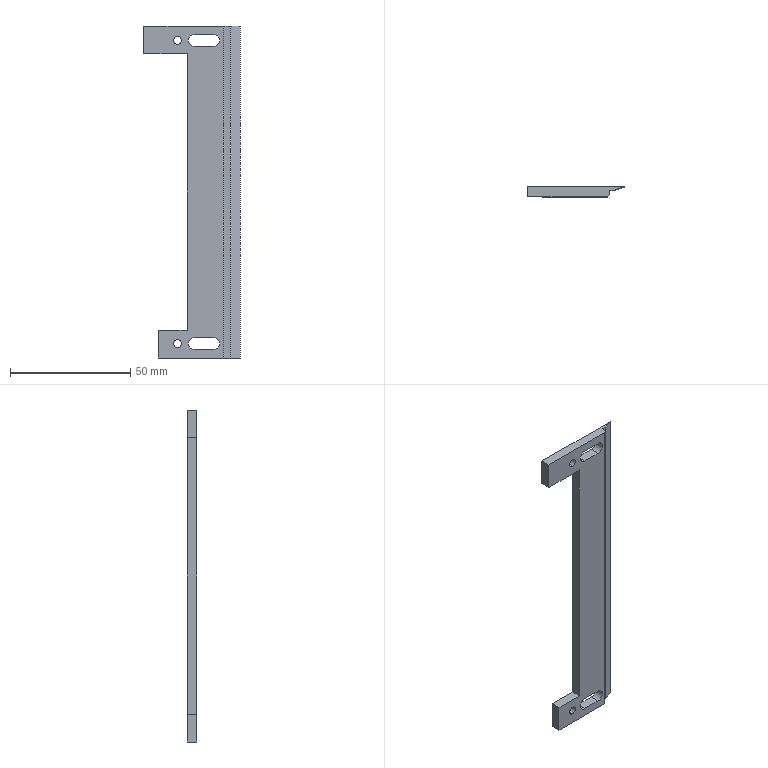Component | SolidWorks | FrameCutterBackingPlate.1-1 | 1 solid | 25 faces | box 40 x 4 x 138 mm | volume 10315 mm3 | plane 17 | cylinder 8 | commonest cylinder face diameters 3.3 x4 5 x4
build123d program:
from build123d import *

# Parameters (mm, degrees)
BOSS_EXTRUDE1_DEPTH   = 4
M4_TAPPED_HOLE1_D     = 3.3
M4_TAPPED_HOLE1_DEPTH = 10.1
M4_TAPPED_HOLE1_TIP   = 0.9914
CUT_EXTRUDE6_DEPTH    = 86.5
CHAMFER1_SIZE         = 1


with BuildPart() as part:
    # Sketch1 → Boss-Extrude1 (new body)
    with BuildSketch(Plane.XY):
        Polygon((-69, 41.921), (69, 41.921), (69, 1.921), (57.5, 1.921), (57.5, 19.921), (-57.5, 19.921), (-57.5, 7.921), (-69, 7.921), align=None)
        with BuildLine():
            Line((-60.5, 30.921), (-60.5, 22.921))
            ThreePointArc((-60.5, 22.921), (-63, 20.421), (-65.5, 22.921))
            Line((-65.5, 22.921), (-65.5, 30.921))
            ThreePointArc((-65.5, 30.921), (-63, 33.421), (-60.5, 30.921))
        make_face(mode=Mode.SUBTRACT)
        with BuildLine():
            Line((65.5, 30.921), (65.5, 22.921))
            ThreePointArc((65.5, 22.921), (63, 20.421), (60.5, 22.921))
            Line((60.5, 22.921), (60.5, 30.921))
            ThreePointArc((60.5, 30.921), (63, 33.421), (65.5, 30.921))
        make_face(mode=Mode.SUBTRACT)
    extrude(amount=BOSS_EXTRUDE1_DEPTH)

    # M4 Tapped Hole1
    with Locations(Plane(origin=(0, 0, 0), x_dir=(-1, 0, 0), z_dir=(0, 0, -1))):
        with Locations((-63, 15.921), (63, 15.921)):
            Hole(M4_TAPPED_HOLE1_D / 2, depth=M4_TAPPED_HOLE1_DEPTH)
            with Locations((0, 0, -(M4_TAPPED_HOLE1_DEPTH + M4_TAPPED_HOLE1_TIP / 2))):  # 118° drill point
                Cone(0, M4_TAPPED_HOLE1_D / 2, M4_TAPPED_HOLE1_TIP, mode=Mode.SUBTRACT)

    # Sketch2 → Cut-Extrude6 (cut, symmetric)
    with BuildSketch(Plane(origin=(0, 0, 0), x_dir=(0, 0, -1), z_dir=(1, 0, 0))):
        Polygon((1.372, 35.921), (-2.7, 35.921), (-2.7, 37.921), (-4, 41.921), (-4, 43.097), (1.372, 43.097), align=None)
    extrude(amount=CUT_EXTRUDE6_DEPTH, both=True, mode=Mode.SUBTRACT)

    # Chamfer1
    chamfer1_edges = [part.edges().sort_by_distance(p)[0] for p in [
        (0, 35.921, 0),
    ]]
    chamfer(chamfer1_edges, length=CHAMFER1_SIZE)


solid = part.part

# Placed as in the assembly
solid = solid.moved(Location((-7.921, 146.5, 0), (-90, 0, -90)))
STEP:
#1=CARTESIAN_POINT('',(0.315,5.925,2.415));
#2=VERTEX_POINT('',#1);
#3=CARTESIAN_POINT('',(0.315,5.925,2.545));
#4=VERTEX_POINT('',#3);
#5=CARTESIAN_POINT('',(0.315,5.925,2.48));
#6=DIRECTION('',(0.,1.,-0.));
#7=DIRECTION('',(0.,0.,1.));
#8=AXIS2_PLACEMENT_3D('',#5,#6,#7);
#9=CIRCLE('',#8,0.06496);
#10=EDGE_CURVE('',#2,#4,#9,.T.);
#11=ORIENTED_EDGE('',*,*,#10,.T.);
#12=CARTESIAN_POINT('',(0.315,5.768,2.545));
#13=VERTEX_POINT('',#12);
#14=CARTESIAN_POINT('',(0.315,5.768,2.545));
#15=DIRECTION('',(-0.,-1.,0.));
#16=VECTOR('',#15,39.37);
#17=LINE('',#14,#16);
#18=EDGE_CURVE('',#4,#13,#17,.T.);
#19=ORIENTED_EDGE('',*,*,#18,.T.);
#20=CARTESIAN_POINT('',(0.315,5.768,2.415));
#21=VERTEX_POINT('',#20);
#22=CARTESIAN_POINT('',(0.315,5.768,2.48));
#23=DIRECTION('',(-0.,-1.,0.));
#24=DIRECTION('',(0.,0.,-1.));
#25=AXIS2_PLACEMENT_3D('',#22,#23,#24);
#26=CIRCLE('',#25,0.06496);
#27=EDGE_CURVE('',#13,#21,#26,.T.);
#28=ORIENTED_EDGE('',*,*,#27,.T.);
#29=CARTESIAN_POINT('',(0.315,5.768,2.415));
#30=DIRECTION('',(-0.,-1.,0.));
#31=VECTOR('',#30,39.37);
#32=LINE('',#29,#31);
#33=EDGE_CURVE('',#2,#21,#32,.T.);
#34=ORIENTED_EDGE('',*,*,#33,.F.);
#35=EDGE_LOOP('',(#11,#19,#28,#34));
#36=FACE_OUTER_BOUND('',#35,.T.);
#37=CARTESIAN_POINT('',(0.315,5.768,2.48));
#38=DIRECTION('',(-0.,-1.,0.));
#39=DIRECTION('',(0.,0.,-1.));
#40=AXIS2_PLACEMENT_3D('',#37,#38,#39);
#41=CYLINDRICAL_SURFACE('',#40,0.06496);
#42=ADVANCED_FACE('',(#36),#41,.F.);
#43=CARTESIAN_POINT('',(0.315,5.925,-2.545));
#44=VERTEX_POINT('',#43);
#45=CARTESIAN_POINT('',(0.315,5.925,-2.415));
#46=VERTEX_POINT('',#45);
#47=CARTESIAN_POINT('',(0.315,5.925,-2.48));
#48=DIRECTION('',(0.,1.,-0.));
#49=DIRECTION('',(0.,0.,1.));
#50=AXIS2_PLACEMENT_3D('',#47,#48,#49);
#51=CIRCLE('',#50,0.06496);
#52=EDGE_CURVE('',#44,#46,#51,.T.);
#53=ORIENTED_EDGE('',*,*,#52,.T.);
#54=CARTESIAN_POINT('',(0.315,5.768,-2.415));
#55=VERTEX_POINT('',#54);
#56=CARTESIAN_POINT('',(0.315,5.768,-2.415));
#57=DIRECTION('',(-0.,-1.,0.));
#58=VECTOR('',#57,39.37);
#59=LINE('',#56,#58);
#60=EDGE_CURVE('',#46,#55,#59,.T.);
#61=ORIENTED_EDGE('',*,*,#60,.T.);
#62=CARTESIAN_POINT('',(0.315,5.768,-2.545));
#63=VERTEX_POINT('',#62);
#64=CARTESIAN_POINT('',(0.315,5.768,-2.48));
#65=DIRECTION('',(-0.,-1.,0.));
#66=DIRECTION('',(0.,0.,-1.));
#67=AXIS2_PLACEMENT_3D('',#64,#65,#66);
#68=CIRCLE('',#67,0.06496);
#69=EDGE_CURVE('',#55,#63,#68,.T.);
#70=ORIENTED_EDGE('',*,*,#69,.T.);
#71=CARTESIAN_POINT('',(0.315,5.768,-2.545));
#72=DIRECTION('',(-0.,-1.,0.));
#73=VECTOR('',#72,39.37);
#74=LINE('',#71,#73);
#75=EDGE_CURVE('',#44,#63,#74,.T.);
#76=ORIENTED_EDGE('',*,*,#75,.F.);
#77=EDGE_LOOP('',(#53,#61,#70,#76));
#78=FACE_OUTER_BOUND('',#77,.T.);
#79=CARTESIAN_POINT('',(0.315,5.768,-2.48));
#80=DIRECTION('',(-0.,-1.,0.));
#81=DIRECTION('',(0.,0.,-1.));
#82=AXIS2_PLACEMENT_3D('',#79,#80,#81);
#83=CYLINDRICAL_SURFACE('',#82,0.06496);
#84=ADVANCED_FACE('',(#78),#83,.F.);
#85=ORIENTED_EDGE('',*,*,#10,.F.);
#86=CARTESIAN_POINT('',(0.315,5.925,2.48));
#87=DIRECTION('',(0.,1.,-0.));
#88=DIRECTION('',(0.,0.,1.));
#89=AXIS2_PLACEMENT_3D('',#86,#87,#88);
#90=CIRCLE('',#89,0.06496);
#91=EDGE_CURVE('',#4,#2,#90,.T.);
#92=ORIENTED_EDGE('',*,*,#91,.F.);
#93=EDGE_LOOP('',(#85,#92));
#94=FACE_BOUND('',#93,.T.);
#95=ORIENTED_EDGE('',*,*,#52,.F.);
#96=CARTESIAN_POINT('',(0.315,5.925,-2.48));
#97=DIRECTION('',(0.,1.,-0.));
#98=DIRECTION('',(0.,0.,1.));
#99=AXIS2_PLACEMENT_3D('',#96,#97,#98);
#100=CIRCLE('',#99,0.06496);
#101=EDGE_CURVE('',#46,#44,#100,.T.);
#102=ORIENTED_EDGE('',*,*,#101,.F.);
#103=EDGE_LOOP('',(#95,#102));
#104=FACE_BOUND('',#103,.T.);
#105=CARTESIAN_POINT('',(0.9055,5.925,-2.579));
#106=VERTEX_POINT('',#105);
#107=CARTESIAN_POINT('',(0.5906,5.925,-2.579));
#108=VERTEX_POINT('',#107);
#109=CARTESIAN_POINT('',(0.9055,5.925,-2.579));
#110=DIRECTION('',(-1.,0.,0.));
#111=VECTOR('',#110,39.37);
#112=LINE('',#109,#111);
#113=EDGE_CURVE('',#106,#108,#112,.T.);
#114=ORIENTED_EDGE('',*,*,#113,.F.);
#115=CARTESIAN_POINT('',(0.9055,5.925,-2.382));
#116=VERTEX_POINT('',#115);
#117=CARTESIAN_POINT('',(0.9055,5.925,-2.48));
#118=DIRECTION('',(0.,1.,-0.));
#119=DIRECTION('',(0.,0.,1.));
#120=AXIS2_PLACEMENT_3D('',#117,#118,#119);
#121=CIRCLE('',#120,0.09843);
#122=EDGE_CURVE('',#116,#106,#121,.T.);
#123=ORIENTED_EDGE('',*,*,#122,.F.);
#124=CARTESIAN_POINT('',(0.5906,5.925,-2.382));
#125=VERTEX_POINT('',#124);
#126=CARTESIAN_POINT('',(0.9055,5.925,-2.382));
#127=DIRECTION('',(1.,-0.,-0.));
#128=VECTOR('',#127,39.37);
#129=LINE('',#126,#128);
#130=EDGE_CURVE('',#125,#116,#129,.T.);
#131=ORIENTED_EDGE('',*,*,#130,.F.);
#132=CARTESIAN_POINT('',(0.5906,5.925,-2.48));
#133=DIRECTION('',(0.,1.,-0.));
#134=DIRECTION('',(0.,0.,1.));
#135=AXIS2_PLACEMENT_3D('',#132,#133,#134);
#136=CIRCLE('',#135,0.09843);
#137=EDGE_CURVE('',#108,#125,#136,.T.);
#138=ORIENTED_EDGE('',*,*,#137,.F.);
#139=EDGE_LOOP('',(#114,#123,#131,#138));
#140=FACE_BOUND('',#139,.T.);
#141=CARTESIAN_POINT('',(1.339,5.925,-2.717));
#142=VERTEX_POINT('',#141);
#143=CARTESIAN_POINT('',(-0.,5.925,-2.717));
#144=VERTEX_POINT('',#143);
#145=CARTESIAN_POINT('',(1.339,5.925,-2.717));
#146=DIRECTION('',(-1.,0.,-0.));
#147=VECTOR('',#146,39.37);
#148=LINE('',#145,#147);
#149=EDGE_CURVE('',#142,#144,#148,.T.);
#150=ORIENTED_EDGE('',*,*,#149,.T.);
#151=CARTESIAN_POINT('',(-0.,5.925,-2.264));
#152=VERTEX_POINT('',#151);
#153=CARTESIAN_POINT('',(-0.,5.925,-2.717));
#154=DIRECTION('',(0.,0.,1.));
#155=VECTOR('',#154,39.37);
#156=LINE('',#153,#155);
#157=EDGE_CURVE('',#144,#152,#156,.T.);
#158=ORIENTED_EDGE('',*,*,#157,.T.);
#159=CARTESIAN_POINT('',(0.4724,5.925,-2.264));
#160=VERTEX_POINT('',#159);
#161=CARTESIAN_POINT('',(-0.,5.925,-2.264));
#162=DIRECTION('',(1.,-0.,-0.));
#163=VECTOR('',#162,39.37);
#164=LINE('',#161,#163);
#165=EDGE_CURVE('',#152,#160,#164,.T.);
#166=ORIENTED_EDGE('',*,*,#165,.T.);
#167=CARTESIAN_POINT('',(0.4724,5.925,2.264));
#168=VERTEX_POINT('',#167);
#169=CARTESIAN_POINT('',(0.4724,5.925,-2.264));
#170=DIRECTION('',(0.,0.,1.));
#171=VECTOR('',#170,39.37);
#172=LINE('',#169,#171);
#173=EDGE_CURVE('',#160,#168,#172,.T.);
#174=ORIENTED_EDGE('',*,*,#173,.T.);
#175=CARTESIAN_POINT('',(-0.2362,5.925,2.264));
#176=VERTEX_POINT('',#175);
#177=CARTESIAN_POINT('',(0.4724,5.925,2.264));
#178=DIRECTION('',(-1.,0.,0.));
#179=VECTOR('',#178,39.37);
#180=LINE('',#177,#179);
#181=EDGE_CURVE('',#168,#176,#180,.T.);
#182=ORIENTED_EDGE('',*,*,#181,.T.);
#183=CARTESIAN_POINT('',(-0.2362,5.925,2.717));
#184=VERTEX_POINT('',#183);
#185=CARTESIAN_POINT('',(-0.2362,5.925,2.264));
#186=DIRECTION('',(0.,0.,1.));
#187=VECTOR('',#186,39.37);
#188=LINE('',#185,#187);
#189=EDGE_CURVE('',#176,#184,#188,.T.);
#190=ORIENTED_EDGE('',*,*,#189,.T.);
#191=CARTESIAN_POINT('',(1.339,5.925,2.717));
#192=VERTEX_POINT('',#191);
#193=CARTESIAN_POINT('',(1.339,5.925,2.717));
#194=DIRECTION('',(1.,-0.,0.));
#195=VECTOR('',#194,39.37);
#196=LINE('',#193,#195);
#197=EDGE_CURVE('',#184,#192,#196,.T.);
#198=ORIENTED_EDGE('',*,*,#197,.T.);
#199=CARTESIAN_POINT('',(1.339,5.925,-2.717));
#200=DIRECTION('',(-0.,-0.,-1.));
#201=VECTOR('',#200,39.37);
#202=LINE('',#199,#201);
#203=EDGE_CURVE('',#192,#142,#202,.T.);
#204=ORIENTED_EDGE('',*,*,#203,.T.);
#205=EDGE_LOOP('',(#150,#158,#166,#174,#182,#190,#198,#204));
#206=FACE_OUTER_BOUND('',#205,.T.);
#207=CARTESIAN_POINT('',(0.9055,5.925,2.382));
#208=VERTEX_POINT('',#207);
#209=CARTESIAN_POINT('',(0.5906,5.925,2.382));
#210=VERTEX_POINT('',#209);
#211=CARTESIAN_POINT('',(0.9055,5.925,2.382));
#212=DIRECTION('',(-1.,0.,0.));
#213=VECTOR('',#212,39.37);
#214=LINE('',#211,#213);
#215=EDGE_CURVE('',#208,#210,#214,.T.);
#216=ORIENTED_EDGE('',*,*,#215,.F.);
#217=CARTESIAN_POINT('',(0.9055,5.925,2.579));
#218=VERTEX_POINT('',#217);
#219=CARTESIAN_POINT('',(0.9055,5.925,2.48));
#220=DIRECTION('',(0.,1.,-0.));
#221=DIRECTION('',(0.,0.,1.));
#222=AXIS2_PLACEMENT_3D('',#219,#220,#221);
#223=CIRCLE('',#222,0.09843);
#224=EDGE_CURVE('',#218,#208,#223,.T.);
#225=ORIENTED_EDGE('',*,*,#224,.F.);
#226=CARTESIAN_POINT('',(0.5906,5.925,2.579));
#227=VERTEX_POINT('',#226);
#228=CARTESIAN_POINT('',(0.9055,5.925,2.579));
#229=DIRECTION('',(1.,-0.,-0.));
#230=VECTOR('',#229,39.37);
#231=LINE('',#228,#230);
#232=EDGE_CURVE('',#227,#218,#231,.T.);
#233=ORIENTED_EDGE('',*,*,#232,.F.);
#234=CARTESIAN_POINT('',(0.5906,5.925,2.48));
#235=DIRECTION('',(0.,1.,-0.));
#236=DIRECTION('',(0.,0.,1.));
#237=AXIS2_PLACEMENT_3D('',#234,#235,#236);
#238=CIRCLE('',#237,0.09843);
#239=EDGE_CURVE('',#210,#227,#238,.T.);
#240=ORIENTED_EDGE('',*,*,#239,.F.);
#241=EDGE_LOOP('',(#216,#225,#233,#240));
#242=FACE_BOUND('',#241,.T.);
#243=CARTESIAN_POINT('',(-0.,5.925,-2.717));
#244=DIRECTION('',(0.,1.,-0.));
#245=DIRECTION('',(0.,0.,1.));
#246=AXIS2_PLACEMENT_3D('',#243,#244,#245);
#247=PLANE('',#246);
#248=ADVANCED_FACE('',(#94,#104,#140,#206,#242),#247,.T.);
#249=CARTESIAN_POINT('',(0.315,5.768,2.48));
#250=DIRECTION('',(-0.,-1.,0.));
#251=DIRECTION('',(0.,0.,-1.));
#252=AXIS2_PLACEMENT_3D('',#249,#250,#251);
#253=CIRCLE('',#252,0.06496);
#254=EDGE_CURVE('',#21,#13,#253,.T.);
#255=ORIENTED_EDGE('',*,*,#254,.F.);
#256=ORIENTED_EDGE('',*,*,#27,.F.);
#257=EDGE_LOOP('',(#255,#256));
#258=FACE_BOUND('',#257,.T.);
#259=CARTESIAN_POINT('',(0.315,5.768,-2.48));
#260=DIRECTION('',(-0.,-1.,0.));
#261=DIRECTION('',(0.,0.,-1.));
#262=AXIS2_PLACEMENT_3D('',#259,#260,#261);
#263=CIRCLE('',#262,0.06496);
#264=EDGE_CURVE('',#63,#55,#263,.T.);
#265=ORIENTED_EDGE('',*,*,#264,.F.);
#266=ORIENTED_EDGE('',*,*,#69,.F.);
#267=EDGE_LOOP('',(#265,#266));
#268=FACE_BOUND('',#267,.T.);
#269=CARTESIAN_POINT('',(0.9055,5.768,-2.382));
#270=VERTEX_POINT('',#269);
#271=CARTESIAN_POINT('',(0.9055,5.768,-2.579));
#272=VERTEX_POINT('',#271);
#273=CARTESIAN_POINT('',(0.9055,5.768,-2.48));
#274=DIRECTION('',(0.,1.,-0.));
#275=DIRECTION('',(0.,0.,1.));
#276=AXIS2_PLACEMENT_3D('',#273,#274,#275);
#277=CIRCLE('',#276,0.09843);
#278=EDGE_CURVE('',#270,#272,#277,.T.);
#279=ORIENTED_EDGE('',*,*,#278,.T.);
#280=CARTESIAN_POINT('',(0.5906,5.768,-2.579));
#281=VERTEX_POINT('',#280);
#282=CARTESIAN_POINT('',(0.9055,5.768,-2.579));
#283=DIRECTION('',(-1.,0.,0.));
#284=VECTOR('',#283,39.37);
#285=LINE('',#282,#284);
#286=EDGE_CURVE('',#272,#281,#285,.T.);
#287=ORIENTED_EDGE('',*,*,#286,.T.);
#288=CARTESIAN_POINT('',(0.5906,5.768,-2.382));
#289=VERTEX_POINT('',#288);
#290=CARTESIAN_POINT('',(0.5906,5.768,-2.48));
#291=DIRECTION('',(0.,1.,-0.));
#292=DIRECTION('',(0.,0.,1.));
#293=AXIS2_PLACEMENT_3D('',#290,#291,#292);
#294=CIRCLE('',#293,0.09843);
#295=EDGE_CURVE('',#281,#289,#294,.T.);
#296=ORIENTED_EDGE('',*,*,#295,.T.);
#297=CARTESIAN_POINT('',(0.9055,5.768,-2.382));
#298=DIRECTION('',(1.,-0.,-0.));
#299=VECTOR('',#298,39.37);
#300=LINE('',#297,#299);
#301=EDGE_CURVE('',#289,#270,#300,.T.);
#302=ORIENTED_EDGE('',*,*,#301,.T.);
#303=EDGE_LOOP('',(#279,#287,#296,#302));
#304=FACE_BOUND('',#303,.T.);
#305=CARTESIAN_POINT('',(1.063,5.768,-2.717));
#306=VERTEX_POINT('',#305);
#307=CARTESIAN_POINT('',(-0.,5.768,-2.717));
#308=VERTEX_POINT('',#307);
#309=CARTESIAN_POINT('',(1.339,5.768,-2.717));
#310=DIRECTION('',(-1.,0.,-0.));
#311=VECTOR('',#310,39.37);
#312=LINE('',#309,#311);
#313=EDGE_CURVE('',#306,#308,#312,.T.);
#314=ORIENTED_EDGE('',*,*,#313,.F.);
#315=CARTESIAN_POINT('',(1.063,5.768,2.717));
#316=VERTEX_POINT('',#315);
#317=CARTESIAN_POINT('',(1.063,5.768,-2.717));
#318=DIRECTION('',(0.,0.,1.));
#319=VECTOR('',#318,39.37);
#320=LINE('',#317,#319);
#321=EDGE_CURVE('',#306,#316,#320,.T.);
#322=ORIENTED_EDGE('',*,*,#321,.T.);
#323=CARTESIAN_POINT('',(-0.2362,5.768,2.717));
#324=VERTEX_POINT('',#323);
#325=CARTESIAN_POINT('',(1.339,5.768,2.717));
#326=DIRECTION('',(1.,-0.,0.));
#327=VECTOR('',#326,39.37);
#328=LINE('',#325,#327);
#329=EDGE_CURVE('',#324,#316,#328,.T.);
#330=ORIENTED_EDGE('',*,*,#329,.F.);
#331=CARTESIAN_POINT('',(-0.2362,5.768,2.264));
#332=VERTEX_POINT('',#331);
#333=CARTESIAN_POINT('',(-0.2362,5.768,2.264));
#334=DIRECTION('',(0.,0.,1.));
#335=VECTOR('',#334,39.37);
#336=LINE('',#333,#335);
#337=EDGE_CURVE('',#332,#324,#336,.T.);
#338=ORIENTED_EDGE('',*,*,#337,.F.);
#339=CARTESIAN_POINT('',(0.4724,5.768,2.264));
#340=VERTEX_POINT('',#339);
#341=CARTESIAN_POINT('',(0.4724,5.768,2.264));
#342=DIRECTION('',(-1.,0.,0.));
#343=VECTOR('',#342,39.37);
#344=LINE('',#341,#343);
#345=EDGE_CURVE('',#340,#332,#344,.T.);
#346=ORIENTED_EDGE('',*,*,#345,.F.);
#347=CARTESIAN_POINT('',(0.4724,5.768,-2.264));
#348=VERTEX_POINT('',#347);
#349=CARTESIAN_POINT('',(0.4724,5.768,-2.264));
#350=DIRECTION('',(0.,0.,1.));
#351=VECTOR('',#350,39.37);
#352=LINE('',#349,#351);
#353=EDGE_CURVE('',#348,#340,#352,.T.);
#354=ORIENTED_EDGE('',*,*,#353,.F.);
#355=CARTESIAN_POINT('',(-0.,5.768,-2.264));
#356=VERTEX_POINT('',#355);
#357=CARTESIAN_POINT('',(-0.,5.768,-2.264));
#358=DIRECTION('',(1.,-0.,-0.));
#359=VECTOR('',#358,39.37);
#360=LINE('',#357,#359);
#361=EDGE_CURVE('',#356,#348,#360,.T.);
#362=ORIENTED_EDGE('',*,*,#361,.F.);
#363=CARTESIAN_POINT('',(-0.,5.768,-2.717));
#364=DIRECTION('',(0.,0.,1.));
#365=VECTOR('',#364,39.37);
#366=LINE('',#363,#365);
#367=EDGE_CURVE('',#308,#356,#366,.T.);
#368=ORIENTED_EDGE('',*,*,#367,.F.);
#369=EDGE_LOOP('',(#314,#322,#330,#338,#346,#354,#362,#368));
#370=FACE_OUTER_BOUND('',#369,.T.);
#371=CARTESIAN_POINT('',(0.9055,5.768,2.579));
#372=VERTEX_POINT('',#371);
#373=CARTESIAN_POINT('',(0.9055,5.768,2.382));
#374=VERTEX_POINT('',#373);
#375=CARTESIAN_POINT('',(0.9055,5.768,2.48));
#376=DIRECTION('',(0.,1.,-0.));
#377=DIRECTION('',(0.,0.,1.));
#378=AXIS2_PLACEMENT_3D('',#375,#376,#377);
#379=CIRCLE('',#378,0.09843);
#380=EDGE_CURVE('',#372,#374,#379,.T.);
#381=ORIENTED_EDGE('',*,*,#380,.T.);
#382=CARTESIAN_POINT('',(0.5906,5.768,2.382));
#383=VERTEX_POINT('',#382);
#384=CARTESIAN_POINT('',(0.9055,5.768,2.382));
#385=DIRECTION('',(-1.,0.,0.));
#386=VECTOR('',#385,39.37);
#387=LINE('',#384,#386);
#388=EDGE_CURVE('',#374,#383,#387,.T.);
#389=ORIENTED_EDGE('',*,*,#388,.T.);
#390=CARTESIAN_POINT('',(0.5906,5.768,2.579));
#391=VERTEX_POINT('',#390);
#392=CARTESIAN_POINT('',(0.5906,5.768,2.48));
#393=DIRECTION('',(0.,1.,-0.));
#394=DIRECTION('',(0.,0.,1.));
#395=AXIS2_PLACEMENT_3D('',#392,#393,#394);
#396=CIRCLE('',#395,0.09843);
#397=EDGE_CURVE('',#383,#391,#396,.T.);
#398=ORIENTED_EDGE('',*,*,#397,.T.);
#399=CARTESIAN_POINT('',(0.9055,5.768,2.579));
#400=DIRECTION('',(1.,-0.,-0.));
#401=VECTOR('',#400,39.37);
#402=LINE('',#399,#401);
#403=EDGE_CURVE('',#391,#372,#402,.T.);
#404=ORIENTED_EDGE('',*,*,#403,.T.);
#405=EDGE_LOOP('',(#381,#389,#398,#404));
#406=FACE_BOUND('',#405,.T.);
#407=CARTESIAN_POINT('',(-0.,5.768,-2.717));
#408=DIRECTION('',(0.,1.,-0.));
#409=DIRECTION('',(0.,0.,1.));
#410=AXIS2_PLACEMENT_3D('',#407,#408,#409);
#411=PLANE('',#410);
#412=ADVANCED_FACE('',(#258,#268,#304,#370,#406),#411,.F.);
#413=CARTESIAN_POINT('',(1.102,5.874,-2.717));
#414=VERTEX_POINT('',#413);
#415=CARTESIAN_POINT('',(1.102,5.807,-2.717));
#416=VERTEX_POINT('',#415);
#417=CARTESIAN_POINT('',(1.102,5.925,-2.717));
#418=DIRECTION('',(-0.,-1.,0.));
#419=VECTOR('',#418,39.37);
#420=LINE('',#417,#419);
#421=EDGE_CURVE('',#414,#416,#420,.T.);
#422=ORIENTED_EDGE('',*,*,#421,.T.);
#423=CARTESIAN_POINT('',(1.063,5.768,-2.717));
#424=DIRECTION('',(-0.7071,-0.7071,-0.));
#425=VECTOR('',#424,39.37);
#426=LINE('',#423,#425);
#427=EDGE_CURVE('',#416,#306,#426,.T.);
#428=ORIENTED_EDGE('',*,*,#427,.T.);
#429=ORIENTED_EDGE('',*,*,#313,.T.);
#430=CARTESIAN_POINT('',(-0.,5.925,-2.717));
#431=DIRECTION('',(-0.,-1.,0.));
#432=VECTOR('',#431,39.37);
#433=LINE('',#430,#432);
#434=EDGE_CURVE('',#144,#308,#433,.T.);
#435=ORIENTED_EDGE('',*,*,#434,.F.);
#436=ORIENTED_EDGE('',*,*,#149,.F.);
#437=CARTESIAN_POINT('',(1.181,5.874,-2.717));
#438=VERTEX_POINT('',#437);
#439=CARTESIAN_POINT('',(1.339,5.925,-2.717));
#440=DIRECTION('',(-0.951,-0.3091,-0.));
#441=VECTOR('',#440,39.37);
#442=LINE('',#439,#441);
#443=EDGE_CURVE('',#142,#438,#442,.T.);
#444=ORIENTED_EDGE('',*,*,#443,.T.);
#445=CARTESIAN_POINT('',(1.339,5.874,-2.717));
#446=DIRECTION('',(-1.,-0.,-0.));
#447=VECTOR('',#446,39.37);
#448=LINE('',#445,#447);
#449=EDGE_CURVE('',#438,#414,#448,.T.);
#450=ORIENTED_EDGE('',*,*,#449,.T.);
#451=EDGE_LOOP('',(#422,#428,#429,#435,#436,#444,#450));
#452=FACE_OUTER_BOUND('',#451,.T.);
#453=CARTESIAN_POINT('',(1.339,5.925,-2.717));
#454=DIRECTION('',(-0.,0.,1.));
#455=DIRECTION('',(1.,-0.,0.));
#456=AXIS2_PLACEMENT_3D('',#453,#454,#455);
#457=PLANE('',#456);
#458=ADVANCED_FACE('',(#452),#457,.F.);
#459=ORIENTED_EDGE('',*,*,#367,.T.);
#460=CARTESIAN_POINT('',(-0.,5.925,-2.264));
#461=DIRECTION('',(-0.,-1.,0.));
#462=VECTOR('',#461,39.37);
#463=LINE('',#460,#462);
#464=EDGE_CURVE('',#152,#356,#463,.T.);
#465=ORIENTED_EDGE('',*,*,#464,.F.);
#466=ORIENTED_EDGE('',*,*,#157,.F.);
#467=ORIENTED_EDGE('',*,*,#434,.T.);
#468=EDGE_LOOP('',(#459,#465,#466,#467));
#469=FACE_OUTER_BOUND('',#468,.T.);
#470=CARTESIAN_POINT('',(-0.,5.925,-2.717));
#471=DIRECTION('',(1.,-0.,-0.));
#472=DIRECTION('',(0.,1.,-0.));
#473=AXIS2_PLACEMENT_3D('',#470,#471,#472);
#474=PLANE('',#473);
#475=ADVANCED_FACE('',(#469),#474,.F.);
#476=ORIENTED_EDGE('',*,*,#361,.T.);
#477=CARTESIAN_POINT('',(0.4724,5.925,-2.264));
#478=DIRECTION('',(-0.,-1.,0.));
#479=VECTOR('',#478,39.37);
#480=LINE('',#477,#479);
#481=EDGE_CURVE('',#160,#348,#480,.T.);
#482=ORIENTED_EDGE('',*,*,#481,.F.);
#483=ORIENTED_EDGE('',*,*,#165,.F.);
#484=ORIENTED_EDGE('',*,*,#464,.T.);
#485=EDGE_LOOP('',(#476,#482,#483,#484));
#486=FACE_OUTER_BOUND('',#485,.T.);
#487=CARTESIAN_POINT('',(-0.,5.925,-2.264));
#488=DIRECTION('',(-0.,-0.,-1.));
#489=DIRECTION('',(0.,1.,-0.));
#490=AXIS2_PLACEMENT_3D('',#487,#488,#489);
#491=PLANE('',#490);
#492=ADVANCED_FACE('',(#486),#491,.F.);
#493=ORIENTED_EDGE('',*,*,#353,.T.);
#494=CARTESIAN_POINT('',(0.4724,5.925,2.264));
#495=DIRECTION('',(-0.,-1.,0.));
#496=VECTOR('',#495,39.37);
#497=LINE('',#494,#496);
#498=EDGE_CURVE('',#168,#340,#497,.T.);
#499=ORIENTED_EDGE('',*,*,#498,.F.);
#500=ORIENTED_EDGE('',*,*,#173,.F.);
#501=ORIENTED_EDGE('',*,*,#481,.T.);
#502=EDGE_LOOP('',(#493,#499,#500,#501));
#503=FACE_OUTER_BOUND('',#502,.T.);
#504=CARTESIAN_POINT('',(0.4724,5.925,-2.264));
#505=DIRECTION('',(1.,-0.,-0.));
#506=DIRECTION('',(0.,1.,-0.));
#507=AXIS2_PLACEMENT_3D('',#504,#505,#506);
#508=PLANE('',#507);
#509=ADVANCED_FACE('',(#503),#508,.F.);
#510=ORIENTED_EDGE('',*,*,#345,.T.);
#511=CARTESIAN_POINT('',(-0.2362,5.925,2.264));
#512=DIRECTION('',(-0.,-1.,0.));
#513=VECTOR('',#512,39.37);
#514=LINE('',#511,#513);
#515=EDGE_CURVE('',#176,#332,#514,.T.);
#516=ORIENTED_EDGE('',*,*,#515,.F.);
#517=ORIENTED_EDGE('',*,*,#181,.F.);
#518=ORIENTED_EDGE('',*,*,#498,.T.);
#519=EDGE_LOOP('',(#510,#516,#517,#518));
#520=FACE_OUTER_BOUND('',#519,.T.);
#521=CARTESIAN_POINT('',(0.4724,5.925,2.264));
#522=DIRECTION('',(0.,0.,1.));
#523=DIRECTION('',(-0.,-1.,0.));
#524=AXIS2_PLACEMENT_3D('',#521,#522,#523);
#525=PLANE('',#524);
#526=ADVANCED_FACE('',(#520),#525,.F.);
#527=ORIENTED_EDGE('',*,*,#337,.T.);
#528=CARTESIAN_POINT('',(-0.2362,5.925,2.717));
#529=DIRECTION('',(-0.,-1.,0.));
#530=VECTOR('',#529,39.37);
#531=LINE('',#528,#530);
#532=EDGE_CURVE('',#184,#324,#531,.T.);
#533=ORIENTED_EDGE('',*,*,#532,.F.);
#534=ORIENTED_EDGE('',*,*,#189,.F.);
#535=ORIENTED_EDGE('',*,*,#515,.T.);
#536=EDGE_LOOP('',(#527,#533,#534,#535));
#537=FACE_OUTER_BOUND('',#536,.T.);
#538=CARTESIAN_POINT('',(-0.2362,5.925,2.264));
#539=DIRECTION('',(1.,-0.,-0.));
#540=DIRECTION('',(-0.,-0.,-1.));
#541=AXIS2_PLACEMENT_3D('',#538,#539,#540);
#542=PLANE('',#541);
#543=ADVANCED_FACE('',(#537),#542,.F.);
#544=ORIENTED_EDGE('',*,*,#329,.T.);
#545=CARTESIAN_POINT('',(1.102,5.807,2.717));
#546=VERTEX_POINT('',#545);
#547=CARTESIAN_POINT('',(1.063,5.768,2.717));
#548=DIRECTION('',(0.7071,0.7071,-0.));
#549=VECTOR('',#548,39.37);
#550=LINE('',#547,#549);
#551=EDGE_CURVE('',#316,#546,#550,.T.);
#552=ORIENTED_EDGE('',*,*,#551,.T.);
#553=CARTESIAN_POINT('',(1.102,5.874,2.717));
#554=VERTEX_POINT('',#553);
#555=CARTESIAN_POINT('',(1.102,5.925,2.717));
#556=DIRECTION('',(0.,1.,-0.));
#557=VECTOR('',#556,39.37);
#558=LINE('',#555,#557);
#559=EDGE_CURVE('',#546,#554,#558,.T.);
#560=ORIENTED_EDGE('',*,*,#559,.T.);
#561=CARTESIAN_POINT('',(1.181,5.874,2.717));
#562=VERTEX_POINT('',#561);
#563=CARTESIAN_POINT('',(1.339,5.874,2.717));
#564=DIRECTION('',(1.,0.,0.));
#565=VECTOR('',#564,39.37);
#566=LINE('',#563,#565);
#567=EDGE_CURVE('',#554,#562,#566,.T.);
#568=ORIENTED_EDGE('',*,*,#567,.T.);
#569=CARTESIAN_POINT('',(1.339,5.925,2.717));
#570=DIRECTION('',(0.951,0.3091,-0.));
#571=VECTOR('',#570,39.37);
#572=LINE('',#569,#571);
#573=EDGE_CURVE('',#562,#192,#572,.T.);
#574=ORIENTED_EDGE('',*,*,#573,.T.);
#575=ORIENTED_EDGE('',*,*,#197,.F.);
#576=ORIENTED_EDGE('',*,*,#532,.T.);
#577=EDGE_LOOP('',(#544,#552,#560,#568,#574,#575,#576));
#578=FACE_OUTER_BOUND('',#577,.T.);
#579=CARTESIAN_POINT('',(1.339,5.925,2.717));
#580=DIRECTION('',(0.,-0.,-1.));
#581=DIRECTION('',(-1.,0.,-0.));
#582=AXIS2_PLACEMENT_3D('',#579,#580,#581);
#583=PLANE('',#582);
#584=ADVANCED_FACE('',(#578),#583,.F.);
#585=ORIENTED_EDGE('',*,*,#278,.F.);
#586=CARTESIAN_POINT('',(0.9055,5.925,-2.382));
#587=DIRECTION('',(-0.,-1.,0.));
#588=VECTOR('',#587,39.37);
#589=LINE('',#586,#588);
#590=EDGE_CURVE('',#116,#270,#589,.T.);
#591=ORIENTED_EDGE('',*,*,#590,.F.);
#592=ORIENTED_EDGE('',*,*,#122,.T.);
#593=CARTESIAN_POINT('',(0.9055,5.925,-2.579));
#594=DIRECTION('',(-0.,-1.,0.));
#595=VECTOR('',#594,39.37);
#596=LINE('',#593,#595);
#597=EDGE_CURVE('',#106,#272,#596,.T.);
#598=ORIENTED_EDGE('',*,*,#597,.T.);
#599=EDGE_LOOP('',(#585,#591,#592,#598));
#600=FACE_OUTER_BOUND('',#599,.T.);
#601=CARTESIAN_POINT('',(0.9055,5.925,-2.48));
#602=DIRECTION('',(-0.,-1.,0.));
#603=DIRECTION('',(0.,0.,-1.));
#604=AXIS2_PLACEMENT_3D('',#601,#602,#603);
#605=CYLINDRICAL_SURFACE('',#604,0.09843);
#606=ADVANCED_FACE('',(#600),#605,.F.);
#607=ORIENTED_EDGE('',*,*,#286,.F.);
#608=ORIENTED_EDGE('',*,*,#597,.F.);
#609=ORIENTED_EDGE('',*,*,#113,.T.);
#610=CARTESIAN_POINT('',(0.5906,5.925,-2.579));
#611=DIRECTION('',(-0.,-1.,0.));
#612=VECTOR('',#611,39.37);
#613=LINE('',#610,#612);
#614=EDGE_CURVE('',#108,#281,#613,.T.);
#615=ORIENTED_EDGE('',*,*,#614,.T.);
#616=EDGE_LOOP('',(#607,#608,#609,#615));
#617=FACE_OUTER_BOUND('',#616,.T.);
#618=CARTESIAN_POINT('',(0.9055,5.925,-2.579));
#619=DIRECTION('',(0.,0.,1.));
#620=DIRECTION('',(-0.,-1.,0.));
#621=AXIS2_PLACEMENT_3D('',#618,#619,#620);
#622=PLANE('',#621);
#623=ADVANCED_FACE('',(#617),#622,.T.);
#624=ORIENTED_EDGE('',*,*,#295,.F.);
#625=ORIENTED_EDGE('',*,*,#614,.F.);
#626=ORIENTED_EDGE('',*,*,#137,.T.);
#627=CARTESIAN_POINT('',(0.5906,5.925,-2.382));
#628=DIRECTION('',(-0.,-1.,0.));
#629=VECTOR('',#628,39.37);
#630=LINE('',#627,#629);
#631=EDGE_CURVE('',#125,#289,#630,.T.);
#632=ORIENTED_EDGE('',*,*,#631,.T.);
#633=EDGE_LOOP('',(#624,#625,#626,#632));
#634=FACE_OUTER_BOUND('',#633,.T.);
#635=CARTESIAN_POINT('',(0.5906,5.925,-2.48));
#636=DIRECTION('',(-0.,-1.,0.));
#637=DIRECTION('',(0.,0.,-1.));
#638=AXIS2_PLACEMENT_3D('',#635,#636,#637);
#639=CYLINDRICAL_SURFACE('',#638,0.09843);
#640=ADVANCED_FACE('',(#634),#639,.F.);
#641=ORIENTED_EDGE('',*,*,#301,.F.);
#642=ORIENTED_EDGE('',*,*,#631,.F.);
#643=ORIENTED_EDGE('',*,*,#130,.T.);
#644=ORIENTED_EDGE('',*,*,#590,.T.);
#645=EDGE_LOOP('',(#641,#642,#643,#644));
#646=FACE_OUTER_BOUND('',#645,.T.);
#647=CARTESIAN_POINT('',(0.9055,5.925,-2.382));
#648=DIRECTION('',(-0.,-0.,-1.));
#649=DIRECTION('',(0.,1.,-0.));
#650=AXIS2_PLACEMENT_3D('',#647,#648,#649);
#651=PLANE('',#650);
#652=ADVANCED_FACE('',(#646),#651,.T.);
#653=ORIENTED_EDGE('',*,*,#380,.F.);
#654=CARTESIAN_POINT('',(0.9055,5.925,2.579));
#655=DIRECTION('',(-0.,-1.,0.));
#656=VECTOR('',#655,39.37);
#657=LINE('',#654,#656);
#658=EDGE_CURVE('',#218,#372,#657,.T.);
#659=ORIENTED_EDGE('',*,*,#658,.F.);
#660=ORIENTED_EDGE('',*,*,#224,.T.);
#661=CARTESIAN_POINT('',(0.9055,5.925,2.382));
#662=DIRECTION('',(-0.,-1.,0.));
#663=VECTOR('',#662,39.37);
#664=LINE('',#661,#663);
#665=EDGE_CURVE('',#208,#374,#664,.T.);
#666=ORIENTED_EDGE('',*,*,#665,.T.);
#667=EDGE_LOOP('',(#653,#659,#660,#666));
#668=FACE_OUTER_BOUND('',#667,.T.);
#669=CARTESIAN_POINT('',(0.9055,5.925,2.48));
#670=DIRECTION('',(-0.,-1.,0.));
#671=DIRECTION('',(0.,0.,-1.));
#672=AXIS2_PLACEMENT_3D('',#669,#670,#671);
#673=CYLINDRICAL_SURFACE('',#672,0.09843);
#674=ADVANCED_FACE('',(#668),#673,.F.);
#675=ORIENTED_EDGE('',*,*,#388,.F.);
#676=ORIENTED_EDGE('',*,*,#665,.F.);
#677=ORIENTED_EDGE('',*,*,#215,.T.);
#678=CARTESIAN_POINT('',(0.5906,5.925,2.382));
#679=DIRECTION('',(-0.,-1.,0.));
#680=VECTOR('',#679,39.37);
#681=LINE('',#678,#680);
#682=EDGE_CURVE('',#210,#383,#681,.T.);
#683=ORIENTED_EDGE('',*,*,#682,.T.);
#684=EDGE_LOOP('',(#675,#676,#677,#683));
#685=FACE_OUTER_BOUND('',#684,.T.);
#686=CARTESIAN_POINT('',(0.9055,5.925,2.382));
#687=DIRECTION('',(0.,0.,1.));
#688=DIRECTION('',(-0.,-1.,0.));
#689=AXIS2_PLACEMENT_3D('',#686,#687,#688);
#690=PLANE('',#689);
#691=ADVANCED_FACE('',(#685),#690,.T.);
#692=ORIENTED_EDGE('',*,*,#397,.F.);
#693=ORIENTED_EDGE('',*,*,#682,.F.);
#694=ORIENTED_EDGE('',*,*,#239,.T.);
#695=CARTESIAN_POINT('',(0.5906,5.925,2.579));
#696=DIRECTION('',(-0.,-1.,0.));
#697=VECTOR('',#696,39.37);
#698=LINE('',#695,#697);
#699=EDGE_CURVE('',#227,#391,#698,.T.);
#700=ORIENTED_EDGE('',*,*,#699,.T.);
#701=EDGE_LOOP('',(#692,#693,#694,#700));
#702=FACE_OUTER_BOUND('',#701,.T.);
#703=CARTESIAN_POINT('',(0.5906,5.925,2.48));
#704=DIRECTION('',(-0.,-1.,0.));
#705=DIRECTION('',(0.,0.,-1.));
#706=AXIS2_PLACEMENT_3D('',#703,#704,#705);
#707=CYLINDRICAL_SURFACE('',#706,0.09843);
#708=ADVANCED_FACE('',(#702),#707,.F.);
#709=ORIENTED_EDGE('',*,*,#403,.F.);
#710=ORIENTED_EDGE('',*,*,#699,.F.);
#711=ORIENTED_EDGE('',*,*,#232,.T.);
#712=ORIENTED_EDGE('',*,*,#658,.T.);
#713=EDGE_LOOP('',(#709,#710,#711,#712));
#714=FACE_OUTER_BOUND('',#713,.T.);
#715=CARTESIAN_POINT('',(0.9055,5.925,2.579));
#716=DIRECTION('',(-0.,-0.,-1.));
#717=DIRECTION('',(0.,1.,-0.));
#718=AXIS2_PLACEMENT_3D('',#715,#716,#717);
#719=PLANE('',#718);
#720=ADVANCED_FACE('',(#714),#719,.T.);
#721=ORIENTED_EDGE('',*,*,#60,.F.);
#722=ORIENTED_EDGE('',*,*,#101,.T.);
#723=ORIENTED_EDGE('',*,*,#75,.T.);
#724=ORIENTED_EDGE('',*,*,#264,.T.);
#725=EDGE_LOOP('',(#721,#722,#723,#724));
#726=FACE_OUTER_BOUND('',#725,.T.);
#727=CARTESIAN_POINT('',(0.315,5.768,-2.48));
#728=DIRECTION('',(-0.,-1.,0.));
#729=DIRECTION('',(0.,0.,-1.));
#730=AXIS2_PLACEMENT_3D('',#727,#728,#729);
#731=CYLINDRICAL_SURFACE('',#730,0.06496);
#732=ADVANCED_FACE('',(#726),#731,.F.);
#733=ORIENTED_EDGE('',*,*,#18,.F.);
#734=ORIENTED_EDGE('',*,*,#91,.T.);
#735=ORIENTED_EDGE('',*,*,#33,.T.);
#736=ORIENTED_EDGE('',*,*,#254,.T.);
#737=EDGE_LOOP('',(#733,#734,#735,#736));
#738=FACE_OUTER_BOUND('',#737,.T.);
#739=CARTESIAN_POINT('',(0.315,5.768,2.48));
#740=DIRECTION('',(-0.,-1.,0.));
#741=DIRECTION('',(0.,0.,-1.));
#742=AXIS2_PLACEMENT_3D('',#739,#740,#741);
#743=CYLINDRICAL_SURFACE('',#742,0.06496);
#744=ADVANCED_FACE('',(#738),#743,.F.);
#745=CARTESIAN_POINT('',(1.181,5.874,-3.406));
#746=DIRECTION('',(0.,0.,1.));
#747=VECTOR('',#746,39.37);
#748=LINE('',#745,#747);
#749=EDGE_CURVE('',#438,#562,#748,.T.);
#750=ORIENTED_EDGE('',*,*,#749,.T.);
#751=ORIENTED_EDGE('',*,*,#567,.F.);
#752=CARTESIAN_POINT('',(1.102,5.874,-3.406));
#753=DIRECTION('',(0.,0.,1.));
#754=VECTOR('',#753,39.37);
#755=LINE('',#752,#754);
#756=EDGE_CURVE('',#414,#554,#755,.T.);
#757=ORIENTED_EDGE('',*,*,#756,.F.);
#758=ORIENTED_EDGE('',*,*,#449,.F.);
#759=EDGE_LOOP('',(#750,#751,#757,#758));
#760=FACE_OUTER_BOUND('',#759,.T.);
#761=CARTESIAN_POINT('',(1.181,5.874,-3.406));
#762=DIRECTION('',(-0.,1.,-0.));
#763=DIRECTION('',(-1.,-0.,0.));
#764=AXIS2_PLACEMENT_3D('',#761,#762,#763);
#765=PLANE('',#764);
#766=ADVANCED_FACE('',(#760),#765,.F.);
#767=ORIENTED_EDGE('',*,*,#559,.F.);
#768=CARTESIAN_POINT('',(1.102,5.807,-3.406));
#769=DIRECTION('',(-0.,-0.,-1.));
#770=VECTOR('',#769,39.37);
#771=LINE('',#768,#770);
#772=EDGE_CURVE('',#546,#416,#771,.T.);
#773=ORIENTED_EDGE('',*,*,#772,.T.);
#774=ORIENTED_EDGE('',*,*,#421,.F.);
#775=ORIENTED_EDGE('',*,*,#756,.T.);
#776=EDGE_LOOP('',(#767,#773,#774,#775));
#777=FACE_OUTER_BOUND('',#776,.T.);
#778=CARTESIAN_POINT('',(1.102,5.714,-3.406));
#779=DIRECTION('',(-1.,0.,0.));
#780=DIRECTION('',(-0.,-1.,0.));
#781=AXIS2_PLACEMENT_3D('',#778,#779,#780);
#782=PLANE('',#781);
#783=ADVANCED_FACE('',(#777),#782,.F.);
#784=ORIENTED_EDGE('',*,*,#203,.F.);
#785=ORIENTED_EDGE('',*,*,#573,.F.);
#786=ORIENTED_EDGE('',*,*,#749,.F.);
#787=ORIENTED_EDGE('',*,*,#443,.F.);
#788=EDGE_LOOP('',(#784,#785,#786,#787));
#789=FACE_OUTER_BOUND('',#788,.T.);
#790=CARTESIAN_POINT('',(1.181,5.874,-3.406));
#791=DIRECTION('',(-0.3091,0.951,-0.));
#792=DIRECTION('',(-0.951,-0.3091,0.));
#793=AXIS2_PLACEMENT_3D('',#790,#791,#792);
#794=PLANE('',#793);
#795=ADVANCED_FACE('',(#789),#794,.F.);
#796=ORIENTED_EDGE('',*,*,#427,.F.);
#797=ORIENTED_EDGE('',*,*,#772,.F.);
#798=ORIENTED_EDGE('',*,*,#551,.F.);
#799=ORIENTED_EDGE('',*,*,#321,.F.);
#800=EDGE_LOOP('',(#796,#797,#798,#799));
#801=FACE_OUTER_BOUND('',#800,.T.);
#802=CARTESIAN_POINT('',(1.063,5.768,-2.717));
#803=DIRECTION('',(-0.7071,0.7071,-0.));
#804=DIRECTION('',(-0.7071,-0.7071,0.));
#805=AXIS2_PLACEMENT_3D('',#802,#803,#804);
#806=PLANE('',#805);
#807=ADVANCED_FACE('',(#801),#806,.F.);
#808=CLOSED_SHELL('',(#42,#84,#248,#412,#458,#475,#492,#509,#526,#543,#584,#606,#623,#640,#652,#674,#691,#708,#720,#732,#744,#766,#783,#795,#807));
#809=MANIFOLD_SOLID_BREP('',#808);
#810=CARTESIAN_POINT('',(0.,0.,0.));
#811=DIRECTION('',(0.,0.,1.));
#812=DIRECTION('',(1.,0.,0.));
#813=AXIS2_PLACEMENT_3D('',#810,#811,#812);
#814=(LENGTH_UNIT()NAMED_UNIT(*)SI_UNIT($,.METRE.));
#815=LENGTH_MEASURE_WITH_UNIT(LENGTH_MEASURE(0.0254),#814);
#816=DIMENSIONAL_EXPONENTS(1.,0.,0.,0.,0.,0.,0.);
#817=(CONVERSION_BASED_UNIT('',#815)LENGTH_UNIT()NAMED_UNIT(#816));
#818=UNCERTAINTY_MEASURE_WITH_UNIT(LENGTH_MEASURE(0.00001),#817,'','');
#819=(NAMED_UNIT(*)PLANE_ANGLE_UNIT()SI_UNIT($,.RADIAN.));
#820=(NAMED_UNIT(*)SI_UNIT($,.STERADIAN.)SOLID_ANGLE_UNIT());
#821=(GEOMETRIC_REPRESENTATION_CONTEXT(3)GLOBAL_UNCERTAINTY_ASSIGNED_CONTEXT((#818))GLOBAL_UNIT_ASSIGNED_CONTEXT((#817,#819,#820))REPRESENTATION_CONTEXT('',''));
#822=ADVANCED_BREP_SHAPE_REPRESENTATION('',(#809,#813),#821);
#823=COLOUR_RGB('',0.7922,0.8196,0.9333);
#824=FILL_AREA_STYLE_COLOUR('',#823);
#825=FILL_AREA_STYLE('',(#824));
#826=SURFACE_STYLE_FILL_AREA(#825);
#827=SURFACE_SIDE_STYLE('',(#826));
#828=SURFACE_STYLE_USAGE(.BOTH.,#827);
#829=PRESENTATION_STYLE_ASSIGNMENT((#828));
#830=STYLED_ITEM('',(#829),#809);
#831=(LENGTH_UNIT()NAMED_UNIT(*)SI_UNIT($,.METRE.));
#832=LENGTH_MEASURE_WITH_UNIT(LENGTH_MEASURE(0.0254),#831);
#833=DIMENSIONAL_EXPONENTS(1.,0.,0.,0.,0.,0.,0.);
#834=(CONVERSION_BASED_UNIT('',#832)LENGTH_UNIT()NAMED_UNIT(#833));
#835=UNCERTAINTY_MEASURE_WITH_UNIT(LENGTH_MEASURE(0.00001),#834,'','');
#836=(NAMED_UNIT(*)PLANE_ANGLE_UNIT()SI_UNIT($,.RADIAN.));
#837=(NAMED_UNIT(*)SI_UNIT($,.STERADIAN.)SOLID_ANGLE_UNIT());
#838=(GEOMETRIC_REPRESENTATION_CONTEXT(3)GLOBAL_UNCERTAINTY_ASSIGNED_CONTEXT((#835))GLOBAL_UNIT_ASSIGNED_CONTEXT((#834,#836,#837))REPRESENTATION_CONTEXT('',''));
#839=MECHANICAL_DESIGN_GEOMETRIC_PRESENTATION_REPRESENTATION('',(#830),#838);
#840=PRESENTATION_LAYER_ASSIGNMENT('','',(#830));